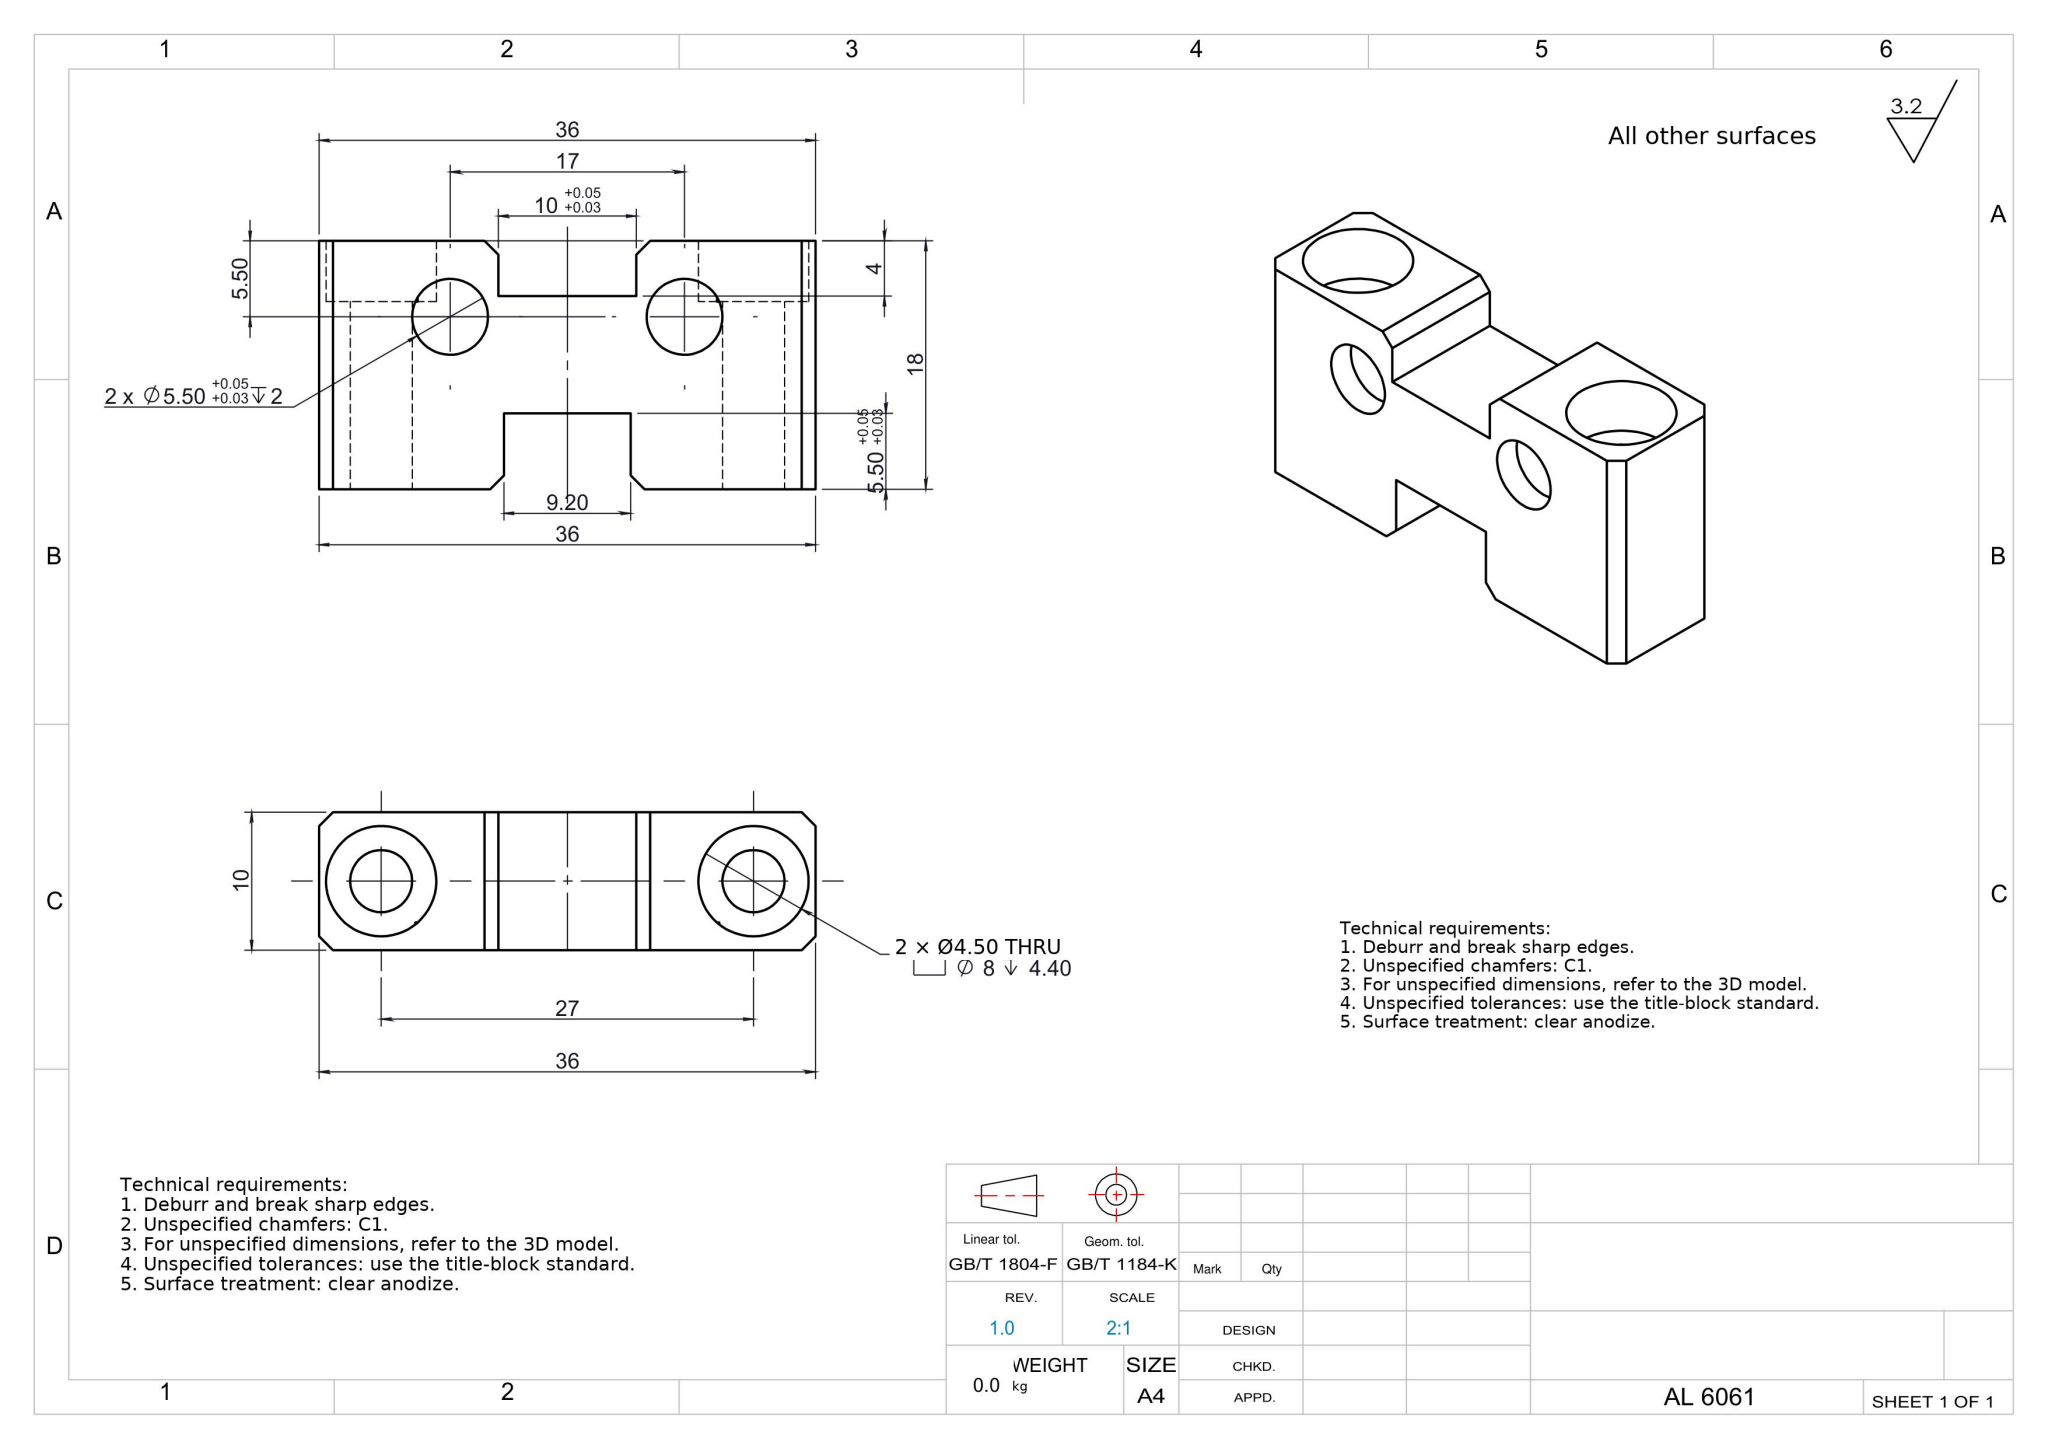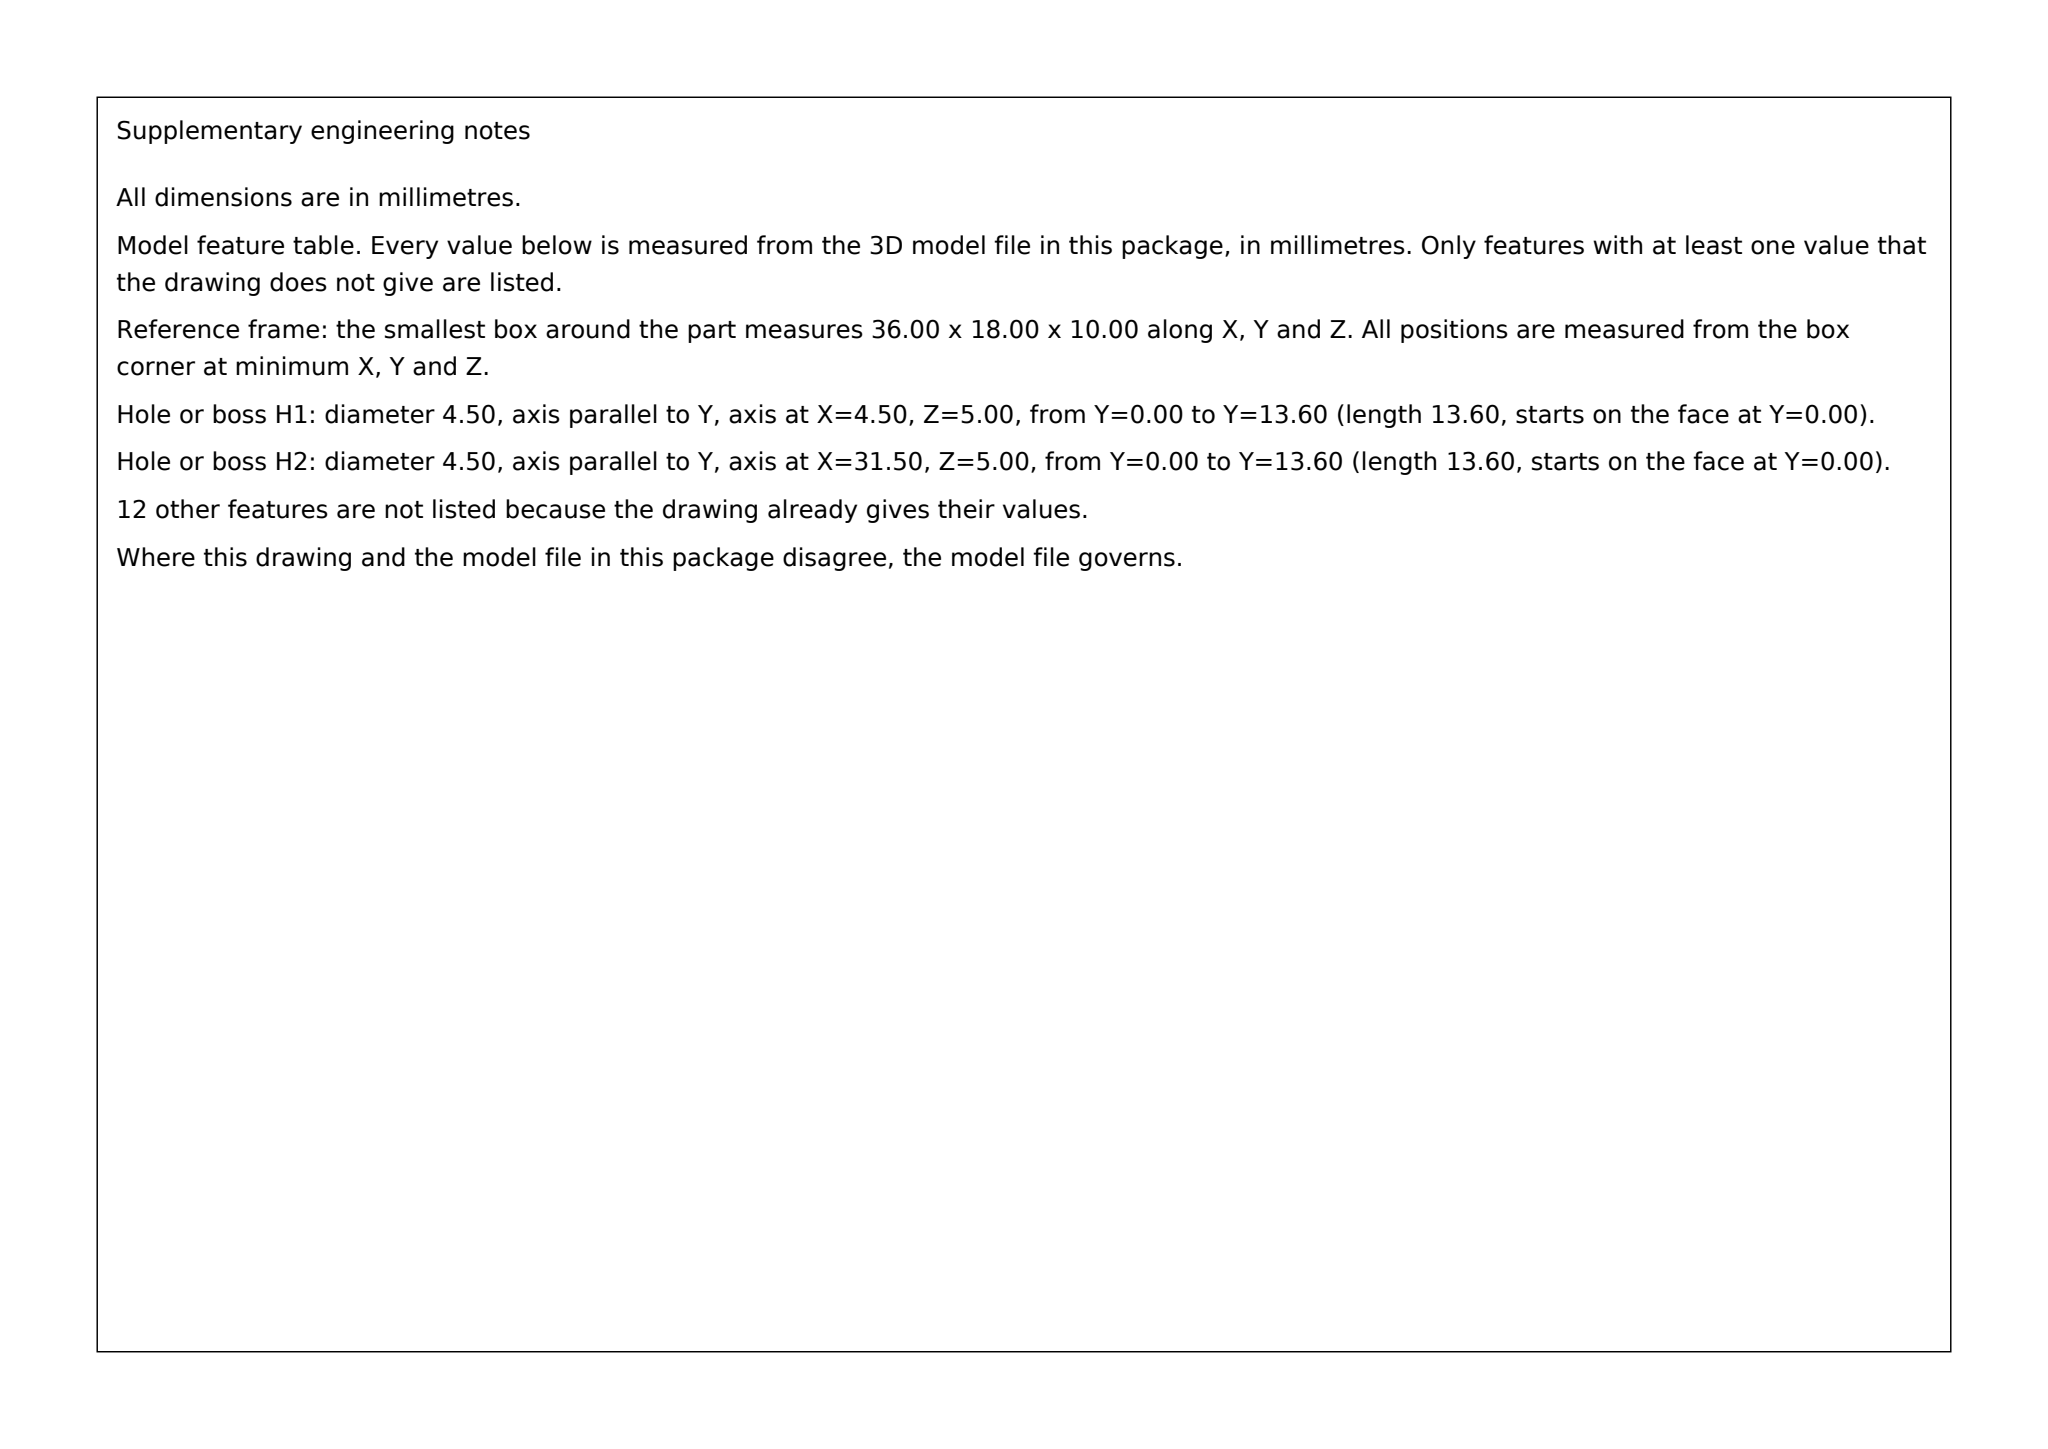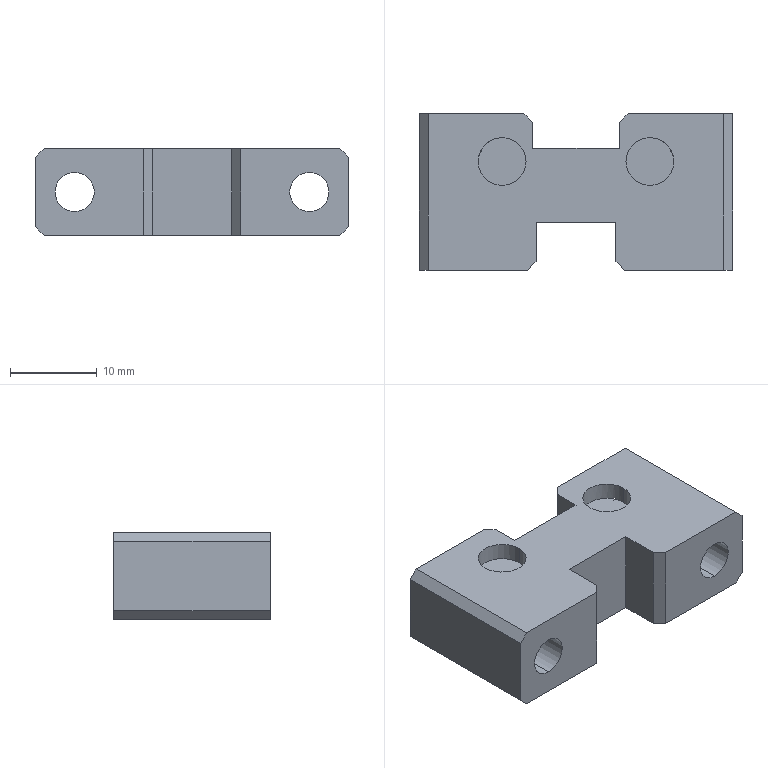Part | SolidWorks | mm | material AL 6061 | 1 solid | 38 faces | box 36 x 18 x 10 mm | volume 4548 mm3 | plane 26 | cylinder 12 | commonest cylinder face diameters 8 x4 4.5 x4 5.5 x4
build123d program:
from build123d import *

# Parameters (mm, degrees)
SKETCH1_W                                       = 26
SKETCH1_H                                       = 18
BOSS_EXTRUDE1_DEPTH                             = 10
SKETCH5_W                                       = 10
SKETCH5_H                                       = 4
CUT_EXTRUDE1_DEPTH                              = 19.708
SKETCH6_R                                       = 2.75
CUT_EXTRUDE2_DEPTH                              = 2
SKETCH7_W                                       = 5
SKETCH7_H                                       = 10
BOSS_EXTRUDE2_DEPTH                             = 18
M4_HEX_SOCKET_HEAD_CAP_SCREW_CBORE2_D           = 4.5
M4_HEX_SOCKET_HEAD_CAP_SCREW_CBORE2_CBORE_D     = 8
M4_HEX_SOCKET_HEAD_CAP_SCREW_CBORE2_CBORE_DEPTH = 4.4
CHAMFER2_SIZE                                   = 1
SKETCH10_W                                      = 9.2
SKETCH10_H                                      = 5.5
CUT_EXTRUDE3_DEPTH                              = 20
CHAMFER3_SIZE                                   = 1


with BuildPart() as part:
    # Sketch1 → Boss-Extrude1 (new body)
    with BuildSketch(Plane.XY):
        Rectangle(SKETCH1_W, SKETCH1_H)
    extrude(amount=BOSS_EXTRUDE1_DEPTH)

    # Sketch5 → Cut-Extrude1 (cut, through all)
    with BuildSketch(Plane(origin=(0, 0, 0), x_dir=(-1, 0, 0), z_dir=(0, 0, -1))):
        with Locations((0, 7)):
            Rectangle(SKETCH5_W, SKETCH5_H)
    extrude(amount=-CUT_EXTRUDE1_DEPTH, mode=Mode.SUBTRACT)

    # Sketch6 → Cut-Extrude2 (cut)
    with BuildSketch(Plane.XY.offset(10)):
        with Locations((-8.5, 3.5)):
            Circle(SKETCH6_R)
        with Locations((8.5, 3.5)):
            Circle(SKETCH6_R)
    extrude(amount=-CUT_EXTRUDE2_DEPTH, mode=Mode.SUBTRACT)

    # Sketch7 → Boss-Extrude2 (add)
    with BuildSketch(Plane.XZ.offset(9)):
        with Locations((-15.5, 5)):
            Rectangle(SKETCH7_W, SKETCH7_H)
        with Locations((15.5, 5)):
            Rectangle(SKETCH7_W, SKETCH7_H)
    extrude(amount=-BOSS_EXTRUDE2_DEPTH)

    # M4 Hex Socket Head Cap Screw CBORE2 (through all)
    with Locations(Plane(origin=(0, 9, 0), x_dir=(1, 0, 0), z_dir=(0, 1, 0))):
        with Locations((-13.5, -5), (13.5, -5)):
            CounterBoreHole(M4_HEX_SOCKET_HEAD_CAP_SCREW_CBORE2_D / 2, M4_HEX_SOCKET_HEAD_CAP_SCREW_CBORE2_CBORE_D / 2, M4_HEX_SOCKET_HEAD_CAP_SCREW_CBORE2_CBORE_DEPTH)

    # Chamfer2
    chamfer2_edges = [part.edges().sort_by_distance(p)[0] for p in [
        (-18, 0, 0),
        (-18, 0, 10),
        (18, 0, 10),
        (18, 0, 0),
    ]]
    chamfer(chamfer2_edges, length=CHAMFER2_SIZE)

    # Sketch10 → Cut-Extrude3 (cut)
    with BuildSketch(Plane.XY.offset(10)):
        with Locations((0, -6.25)):
            Rectangle(SKETCH10_W, SKETCH10_H)
    extrude(amount=-CUT_EXTRUDE3_DEPTH, mode=Mode.SUBTRACT)

    # Chamfer3
    chamfer3_edges = [part.edges().sort_by_distance(p)[0] for p in [
        (-4.6, -9, 5),
        (4.6, -9, 5),
        (5, 9, 5),
        (-5, 9, 5),
    ]]
    chamfer(chamfer3_edges, length=CHAMFER3_SIZE)


solid = part.part